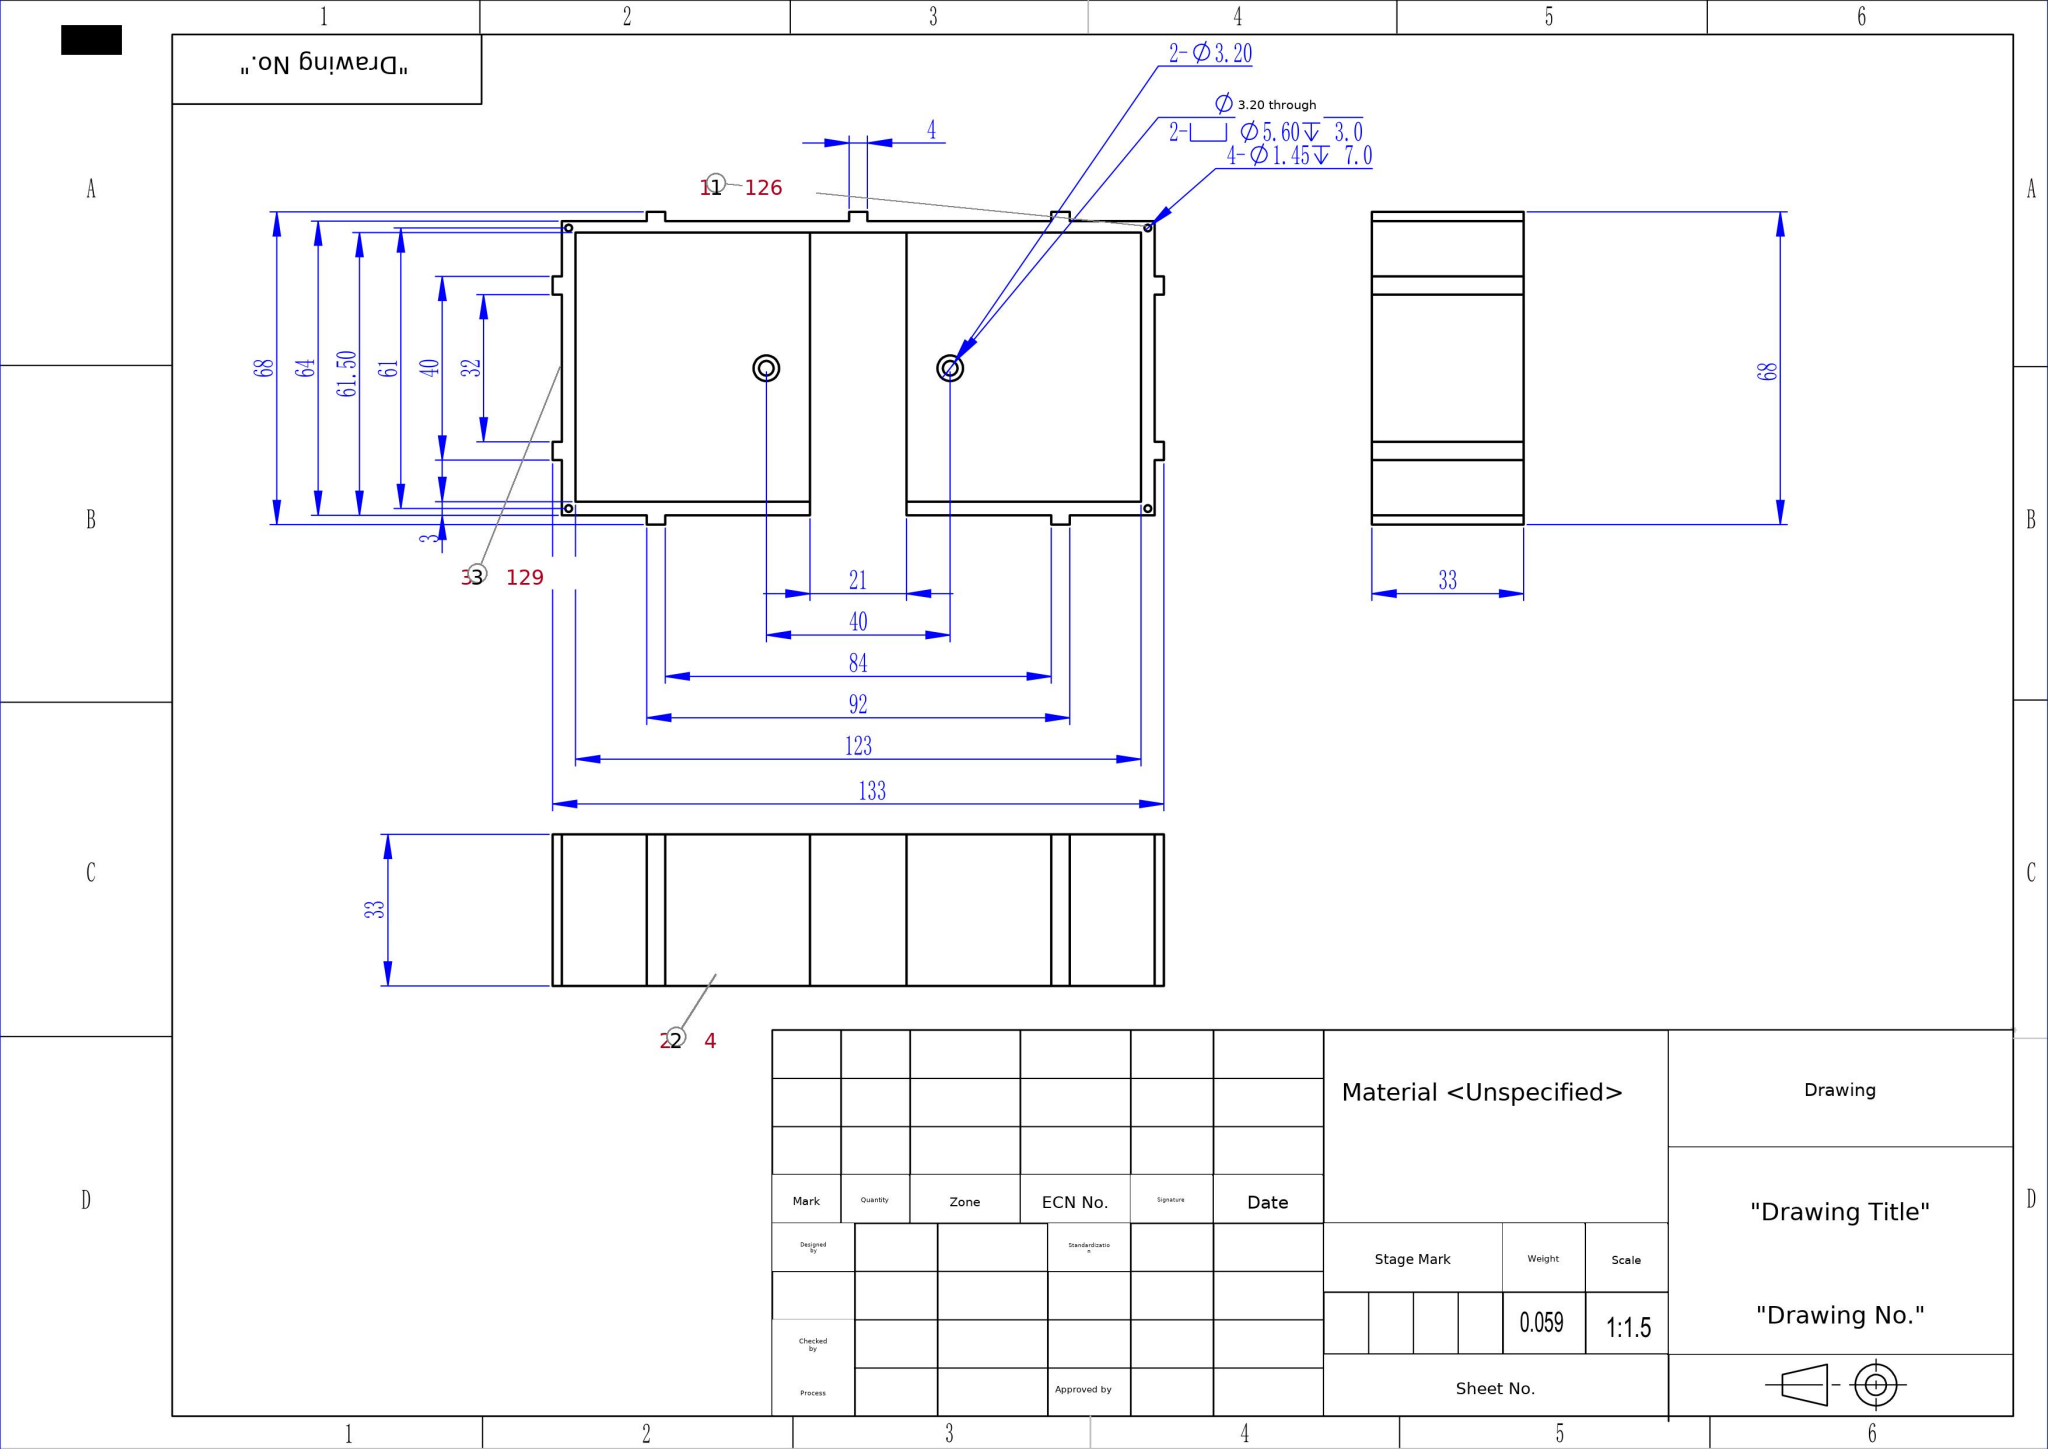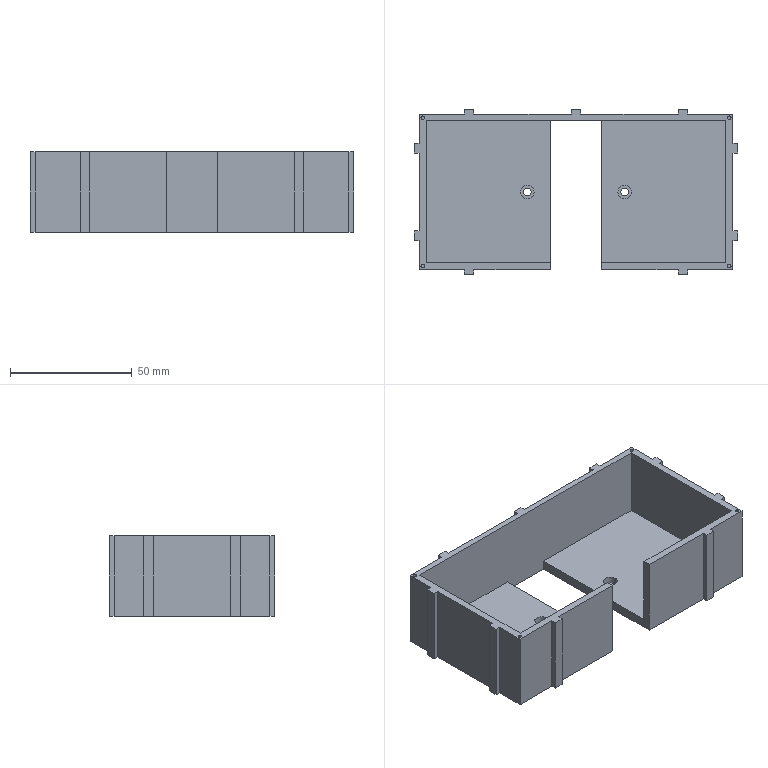Part | SolidWorks | mm | 1 solid | 74 faces | box 133 x 68 x 33 mm | volume 58951 mm3 | plane 58 | cylinder 16 | commonest cylinder face diameters 1.45 x8 5.6 x4 3.2 x4
build123d program:
from build123d import *

# Parameters (mm, degrees)
MODEL_R             = 1.6
BOSS_EXTRUDE1_DEPTH = 4
CUT_EXTRUDE1_START  = -3
SKETCH2_R           = 2.8
SKETCH2_R_2         = 1.6
CUT_EXTRUDE1_DEPTH  = 3
BOSS_EXTRUDE2_DEPTH = 29
SKETCH6_R           = 0.725
CUT_EXTRUDE2_DEPTH  = 7


with BuildPart() as part:
    # Model → Boss-Extrude1 (new body)
    with BuildSketch(Plane.XY):
        Polygon((257.556, 185.18), (276.056, 185.18), (276.056, 187.18), (280.056, 187.18), (280.056, 185.18), (320.056, 185.18), (320.056, 187.18), (324.056, 187.18), (324.056, 185.18), (364.056, 185.18), (364.056, 187.18), (368.056, 187.18), (368.056, 185.18), (386.556, 185.18), (386.556, 173.18), (388.556, 173.18), (388.556, 169.18), (386.556, 169.18), (386.556, 137.18), (388.556, 137.18), (388.556, 133.18), (386.556, 133.18), (386.556, 121.18), (368.056, 121.18), (368.056, 119.18), (364.056, 119.18), (364.056, 121.18), (332.556, 121.18), (332.556, 182.68), (311.556, 182.68), (311.556, 121.18), (280.056, 121.18), (280.056, 119.18), (276.056, 119.18), (276.056, 121.18), (257.556, 121.18), (257.556, 133.18), (255.556, 133.18), (255.556, 137.18), (257.556, 137.18), (257.556, 169.18), (255.556, 169.18), (255.556, 173.18), (257.556, 173.18), align=None)
        with Locations((342.056, 153.18)):
            Circle(MODEL_R, mode=Mode.SUBTRACT)
        with Locations((302.056, 153.18)):
            Circle(MODEL_R, mode=Mode.SUBTRACT)
    extrude(amount=BOSS_EXTRUDE1_DEPTH)

    # Sketch2 → Cut-Extrude1 (cut)
    # profile 1 of 2: a face of its own
    with BuildSketch(Plane.XY.offset(4).offset(CUT_EXTRUDE1_START)):
        with Locations((302.056, 153.18)):
            Circle(SKETCH2_R)
        with Locations((302.056, 153.18)):
            Circle(SKETCH2_R_2, mode=Mode.SUBTRACT)
    # profile 2 of 2: a face of its own
    with BuildSketch(Plane.XY.offset(4).offset(CUT_EXTRUDE1_START)):
        with Locations((342.056, 153.18)):
            Circle(SKETCH2_R)
        with Locations((342.056, 153.18)):
            Circle(SKETCH2_R_2, mode=Mode.SUBTRACT)
    extrude(amount=CUT_EXTRUDE1_DEPTH, mode=Mode.SUBTRACT)

    # Sketch3 → Boss-Extrude2 (add)
    with BuildSketch(Plane.XY.offset(4)):
        Polygon((260.556, 182.68), (260.556, 124.18), (311.556, 124.18), (311.556, 121.18), (280.056, 121.18), (280.056, 119.18), (276.056, 119.18), (276.056, 121.18), (257.556, 121.18), (257.556, 133.18), (255.556, 133.18), (255.556, 137.18), (257.556, 137.18), (257.556, 169.18), (255.556, 169.18), (255.556, 173.18), (257.556, 173.18), (257.556, 185.18), (276.056, 185.18), (276.056, 187.18), (280.056, 187.18), (280.056, 185.18), (320.056, 185.18), (320.056, 187.18), (324.056, 187.18), (324.056, 185.18), (364.056, 185.18), (364.056, 187.18), (368.056, 187.18), (368.056, 185.18), (386.556, 185.18), (386.556, 173.18), (388.556, 173.18), (388.556, 169.18), (386.556, 169.18), (386.556, 137.18), (388.556, 137.18), (388.556, 133.18), (386.556, 133.18), (386.556, 121.18), (368.056, 121.18), (368.056, 119.18), (364.056, 119.18), (364.056, 121.18), (332.556, 121.18), (332.556, 124.18), (383.556, 124.18), (383.556, 182.68), align=None)
    extrude(amount=BOSS_EXTRUDE2_DEPTH)

    # Sketch6 → Cut-Extrude2 (cut)
    with BuildSketch(Plane.XY.offset(33)):
        with Locations((259.056, 183.68)):
            Circle(SKETCH6_R)
        with Locations((385.056, 183.68)):
            Circle(SKETCH6_R)
        with Locations((385.056, 122.68)):
            Circle(SKETCH6_R)
        with Locations((259.056, 122.68)):
            Circle(SKETCH6_R)
    extrude(amount=-CUT_EXTRUDE2_DEPTH, mode=Mode.SUBTRACT)


solid = part.part